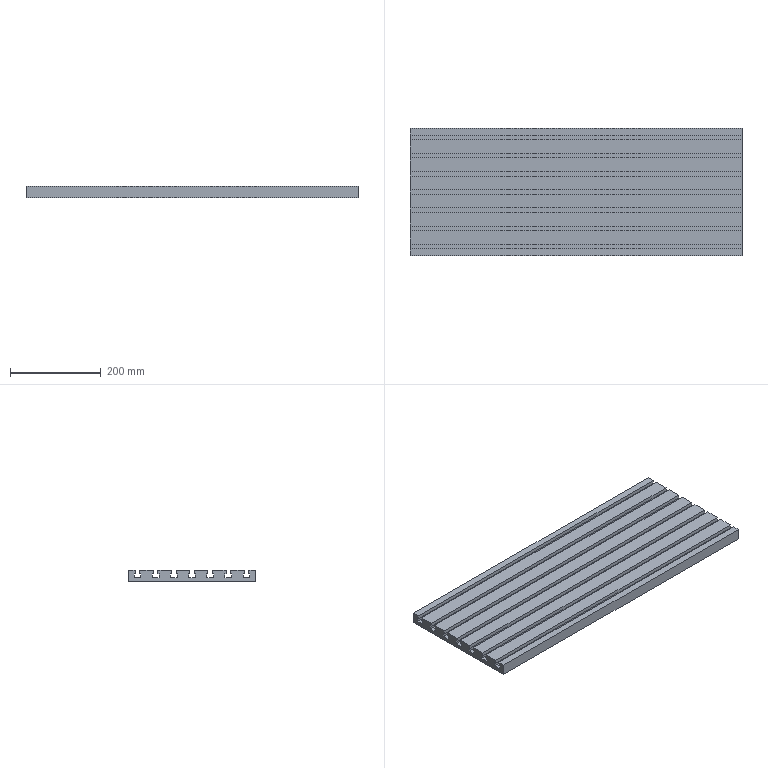Component | NX | MACHINE_TOOL_PLATFORM | 1 solid | 62 faces | volume 4088000 mm3 | plane 62